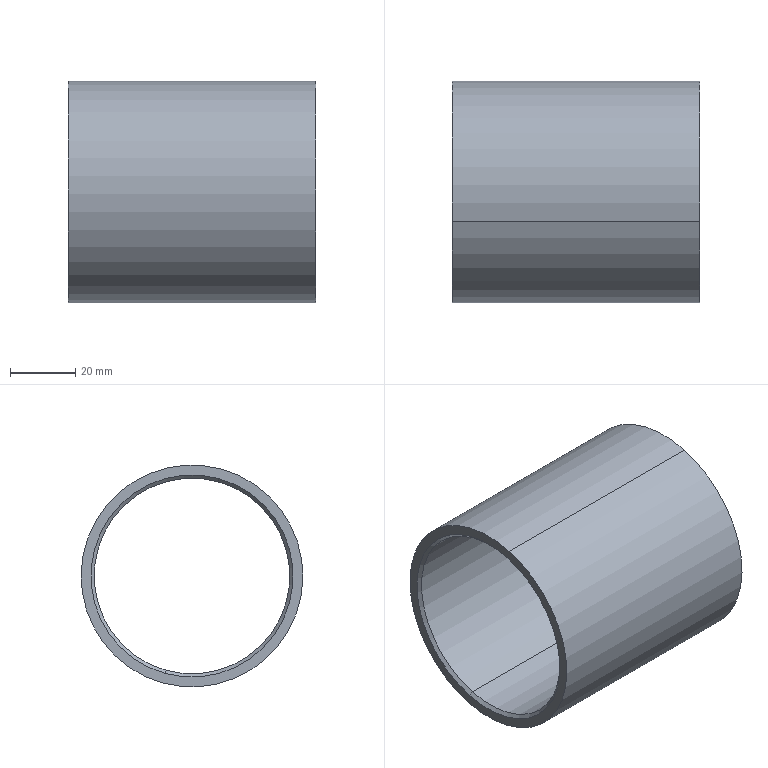Component | SolidWorks | SpindleSleeve3-1 | 1 solid | 10 faces | box 76 x 68 x 68 mm | volume 60932 mm3 | cone 4 | cylinder 4 | plane 2 | commonest cylinder face diameters 60 x2 68 x2
build123d program:
from build123d import *

# Parameters (mm, degrees)
SKETCH1_R           = 34
SKETCH1_R_2         = 30
BOSS_EXTRUDE1_DEPTH = 38
CHAMFER1_SIZE       = 1


with BuildPart() as part:
    # Sketch1 → Boss-Extrude1 (new, symmetric)
    with BuildSketch(Plane(origin=(0, 0, 0), x_dir=(1, 0, 0), z_dir=(0, 1, 0))):
        with Locations(Location((0, 0, 0), (0, 0, 270))):
            Circle(SKETCH1_R)
        with Locations(Location((0, 0, 0), (0, 0, 270))):
            Circle(SKETCH1_R_2, mode=Mode.SUBTRACT)
    extrude(amount=BOSS_EXTRUDE1_DEPTH, both=True)

    # Chamfer1
    chamfer1_edges = [part.edges().sort_by_distance(p)[0] for p in [
        (0, -38, -30),
        (0, 38, -30),
    ]]
    chamfer(chamfer1_edges, length=CHAMFER1_SIZE)


solid = part.part

# Placed as in the assembly
solid = solid.moved(Location((-713.197, 34.532, 0), (0, 0, 90)))
STEP:
#1=CARTESIAN_POINT('',(-26.622,1.671,-1.139));
#2=VERTEX_POINT('',#1);
#3=CARTESIAN_POINT('',(-26.622,1.048,1.139));
#4=VERTEX_POINT('',#3);
#5=CARTESIAN_POINT('',(-26.622,1.36,0.));
#6=DIRECTION('',(1.,0.,0.));
#7=DIRECTION('',(0.,0.2635,-0.9647));
#8=AXIS2_PLACEMENT_3D('',#5,#6,#7);
#9=CIRCLE('',#8,1.181);
#10=EDGE_CURVE('',#2,#4,#9,.T.);
#11=ORIENTED_EDGE('',*,*,#10,.F.);
#12=CARTESIAN_POINT('',(-26.583,1.681,-1.177));
#13=VERTEX_POINT('',#12);
#14=CARTESIAN_POINT('',(-26.583,1.681,-1.177));
#15=DIRECTION('',(0.7071,0.1863,-0.6821));
#16=VECTOR('',#15,39.37);
#17=LINE('',#14,#16);
#18=EDGE_CURVE('',#2,#13,#17,.T.);
#19=ORIENTED_EDGE('',*,*,#18,.T.);
#20=CARTESIAN_POINT('',(-26.583,1.038,1.177));
#21=VERTEX_POINT('',#20);
#22=CARTESIAN_POINT('',(-26.583,1.36,0.));
#23=DIRECTION('',(-1.,0.,0.));
#24=DIRECTION('',(0.,0.2635,-0.9647));
#25=AXIS2_PLACEMENT_3D('',#22,#23,#24);
#26=CIRCLE('',#25,1.22);
#27=EDGE_CURVE('',#21,#13,#26,.T.);
#28=ORIENTED_EDGE('',*,*,#27,.F.);
#29=CARTESIAN_POINT('',(-26.583,1.038,1.177));
#30=DIRECTION('',(0.7071,-0.1863,0.6821));
#31=VECTOR('',#30,39.37);
#32=LINE('',#29,#31);
#33=EDGE_CURVE('',#4,#21,#32,.T.);
#34=ORIENTED_EDGE('',*,*,#33,.F.);
#35=EDGE_LOOP('',(#11,#19,#28,#34));
#36=FACE_OUTER_BOUND('',#35,.T.);
#37=CARTESIAN_POINT('',(-26.583,1.36,0.));
#38=DIRECTION('',(1.,0.,0.));
#39=DIRECTION('',(0.,-0.2635,0.9647));
#40=AXIS2_PLACEMENT_3D('',#37,#38,#39);
#41=CONICAL_SURFACE('',#40,1.22,0.7854);
#42=ADVANCED_FACE('',(#36),#41,.F.);
#43=CARTESIAN_POINT('',(-29.535,1.048,1.139));
#44=VERTEX_POINT('',#43);
#45=CARTESIAN_POINT('',(-29.535,1.671,-1.139));
#46=VERTEX_POINT('',#45);
#47=CARTESIAN_POINT('',(-29.535,1.36,0.));
#48=DIRECTION('',(-1.,0.,0.));
#49=DIRECTION('',(0.,0.2635,-0.9647));
#50=AXIS2_PLACEMENT_3D('',#47,#48,#49);
#51=CIRCLE('',#50,1.181);
#52=EDGE_CURVE('',#44,#46,#51,.T.);
#53=ORIENTED_EDGE('',*,*,#52,.F.);
#54=CARTESIAN_POINT('',(-29.575,1.038,1.177));
#55=VERTEX_POINT('',#54);
#56=CARTESIAN_POINT('',(-29.535,1.048,1.139));
#57=DIRECTION('',(-0.7071,-0.1863,0.6821));
#58=VECTOR('',#57,39.37);
#59=LINE('',#56,#58);
#60=EDGE_CURVE('',#44,#55,#59,.T.);
#61=ORIENTED_EDGE('',*,*,#60,.T.);
#62=CARTESIAN_POINT('',(-29.575,1.681,-1.177));
#63=VERTEX_POINT('',#62);
#64=CARTESIAN_POINT('',(-29.575,1.36,0.));
#65=DIRECTION('',(1.,0.,0.));
#66=DIRECTION('',(0.,0.2635,-0.9647));
#67=AXIS2_PLACEMENT_3D('',#64,#65,#66);
#68=CIRCLE('',#67,1.22);
#69=EDGE_CURVE('',#63,#55,#68,.T.);
#70=ORIENTED_EDGE('',*,*,#69,.F.);
#71=CARTESIAN_POINT('',(-29.535,1.671,-1.139));
#72=DIRECTION('',(-0.7071,0.1863,-0.6821));
#73=VECTOR('',#72,39.37);
#74=LINE('',#71,#73);
#75=EDGE_CURVE('',#46,#63,#74,.T.);
#76=ORIENTED_EDGE('',*,*,#75,.F.);
#77=EDGE_LOOP('',(#53,#61,#70,#76));
#78=FACE_OUTER_BOUND('',#77,.T.);
#79=CARTESIAN_POINT('',(-29.535,1.36,0.));
#80=DIRECTION('',(-1.,0.,0.));
#81=DIRECTION('',(0.,0.2635,-0.9647));
#82=AXIS2_PLACEMENT_3D('',#79,#80,#81);
#83=CONICAL_SURFACE('',#82,1.181,0.7854);
#84=ADVANCED_FACE('',(#78),#83,.F.);
#85=ORIENTED_EDGE('',*,*,#52,.T.);
#86=CARTESIAN_POINT('',(-29.575,1.671,-1.139));
#87=DIRECTION('',(1.,0.,0.));
#88=VECTOR('',#87,39.37);
#89=LINE('',#86,#88);
#90=EDGE_CURVE('',#46,#2,#89,.T.);
#91=ORIENTED_EDGE('',*,*,#90,.T.);
#92=ORIENTED_EDGE('',*,*,#10,.T.);
#93=CARTESIAN_POINT('',(-29.575,1.048,1.139));
#94=DIRECTION('',(1.,0.,0.));
#95=VECTOR('',#94,39.37);
#96=LINE('',#93,#95);
#97=EDGE_CURVE('',#44,#4,#96,.T.);
#98=ORIENTED_EDGE('',*,*,#97,.F.);
#99=EDGE_LOOP('',(#85,#91,#92,#98));
#100=FACE_OUTER_BOUND('',#99,.T.);
#101=CARTESIAN_POINT('',(-29.575,1.36,0.));
#102=DIRECTION('',(1.,0.,0.));
#103=DIRECTION('',(0.,-0.2635,0.9647));
#104=AXIS2_PLACEMENT_3D('',#101,#102,#103);
#105=CYLINDRICAL_SURFACE('',#104,1.181);
#106=ADVANCED_FACE('',(#100),#105,.F.);
#107=CARTESIAN_POINT('',(-29.575,1.712,-1.291));
#108=VERTEX_POINT('',#107);
#109=CARTESIAN_POINT('',(-29.575,1.007,1.291));
#110=VERTEX_POINT('',#109);
#111=CARTESIAN_POINT('',(-29.575,1.36,0.));
#112=DIRECTION('',(-1.,0.,0.));
#113=DIRECTION('',(0.,0.2635,-0.9647));
#114=AXIS2_PLACEMENT_3D('',#111,#112,#113);
#115=CIRCLE('',#114,1.339);
#116=EDGE_CURVE('',#108,#110,#115,.T.);
#117=ORIENTED_EDGE('',*,*,#116,.F.);
#118=CARTESIAN_POINT('',(-26.583,1.712,-1.291));
#119=VERTEX_POINT('',#118);
#120=CARTESIAN_POINT('',(-29.575,1.712,-1.291));
#121=DIRECTION('',(1.,0.,0.));
#122=VECTOR('',#121,39.37);
#123=LINE('',#120,#122);
#124=EDGE_CURVE('',#108,#119,#123,.T.);
#125=ORIENTED_EDGE('',*,*,#124,.T.);
#126=CARTESIAN_POINT('',(-26.583,1.007,1.291));
#127=VERTEX_POINT('',#126);
#128=CARTESIAN_POINT('',(-26.583,1.36,0.));
#129=DIRECTION('',(-1.,0.,0.));
#130=DIRECTION('',(0.,0.2635,-0.9647));
#131=AXIS2_PLACEMENT_3D('',#128,#129,#130);
#132=CIRCLE('',#131,1.339);
#133=EDGE_CURVE('',#119,#127,#132,.T.);
#134=ORIENTED_EDGE('',*,*,#133,.T.);
#135=CARTESIAN_POINT('',(-29.575,1.007,1.291));
#136=DIRECTION('',(1.,0.,0.));
#137=VECTOR('',#136,39.37);
#138=LINE('',#135,#137);
#139=EDGE_CURVE('',#110,#127,#138,.T.);
#140=ORIENTED_EDGE('',*,*,#139,.F.);
#141=EDGE_LOOP('',(#117,#125,#134,#140));
#142=FACE_OUTER_BOUND('',#141,.T.);
#143=CARTESIAN_POINT('',(-29.575,1.36,0.));
#144=DIRECTION('',(1.,0.,0.));
#145=DIRECTION('',(0.,-0.2635,0.9647));
#146=AXIS2_PLACEMENT_3D('',#143,#144,#145);
#147=CYLINDRICAL_SURFACE('',#146,1.339);
#148=ADVANCED_FACE('',(#142),#147,.T.);
#149=ORIENTED_EDGE('',*,*,#69,.T.);
#150=CARTESIAN_POINT('',(-29.575,1.36,0.));
#151=DIRECTION('',(1.,0.,0.));
#152=DIRECTION('',(0.,0.2635,-0.9647));
#153=AXIS2_PLACEMENT_3D('',#150,#151,#152);
#154=CIRCLE('',#153,1.22);
#155=EDGE_CURVE('',#55,#63,#154,.T.);
#156=ORIENTED_EDGE('',*,*,#155,.T.);
#157=EDGE_LOOP('',(#149,#156));
#158=FACE_BOUND('',#157,.T.);
#159=CARTESIAN_POINT('',(-29.575,1.36,0.));
#160=DIRECTION('',(-1.,0.,0.));
#161=DIRECTION('',(0.,0.2635,-0.9647));
#162=AXIS2_PLACEMENT_3D('',#159,#160,#161);
#163=CIRCLE('',#162,1.339);
#164=EDGE_CURVE('',#110,#108,#163,.T.);
#165=ORIENTED_EDGE('',*,*,#164,.T.);
#166=ORIENTED_EDGE('',*,*,#116,.T.);
#167=EDGE_LOOP('',(#165,#166));
#168=FACE_OUTER_BOUND('',#167,.T.);
#169=CARTESIAN_POINT('',(-29.575,1.36,0.));
#170=DIRECTION('',(-1.,0.,0.));
#171=DIRECTION('',(0.,0.2635,-0.9647));
#172=AXIS2_PLACEMENT_3D('',#169,#170,#171);
#173=PLANE('',#172);
#174=ADVANCED_FACE('',(#158,#168),#173,.T.);
#175=ORIENTED_EDGE('',*,*,#27,.T.);
#176=CARTESIAN_POINT('',(-26.583,1.36,0.));
#177=DIRECTION('',(-1.,0.,0.));
#178=DIRECTION('',(0.,0.2635,-0.9647));
#179=AXIS2_PLACEMENT_3D('',#176,#177,#178);
#180=CIRCLE('',#179,1.22);
#181=EDGE_CURVE('',#13,#21,#180,.T.);
#182=ORIENTED_EDGE('',*,*,#181,.T.);
#183=EDGE_LOOP('',(#175,#182));
#184=FACE_BOUND('',#183,.T.);
#185=CARTESIAN_POINT('',(-26.583,1.36,0.));
#186=DIRECTION('',(-1.,0.,0.));
#187=DIRECTION('',(0.,0.2635,-0.9647));
#188=AXIS2_PLACEMENT_3D('',#185,#186,#187);
#189=CIRCLE('',#188,1.339);
#190=EDGE_CURVE('',#127,#119,#189,.T.);
#191=ORIENTED_EDGE('',*,*,#190,.F.);
#192=ORIENTED_EDGE('',*,*,#133,.F.);
#193=EDGE_LOOP('',(#191,#192));
#194=FACE_OUTER_BOUND('',#193,.T.);
#195=CARTESIAN_POINT('',(-26.583,1.36,0.));
#196=DIRECTION('',(-1.,0.,0.));
#197=DIRECTION('',(0.,0.2635,-0.9647));
#198=AXIS2_PLACEMENT_3D('',#195,#196,#197);
#199=PLANE('',#198);
#200=ADVANCED_FACE('',(#184,#194),#199,.F.);
#201=ORIENTED_EDGE('',*,*,#124,.F.);
#202=ORIENTED_EDGE('',*,*,#164,.F.);
#203=ORIENTED_EDGE('',*,*,#139,.T.);
#204=ORIENTED_EDGE('',*,*,#190,.T.);
#205=EDGE_LOOP('',(#201,#202,#203,#204));
#206=FACE_OUTER_BOUND('',#205,.T.);
#207=CARTESIAN_POINT('',(-29.575,1.36,0.));
#208=DIRECTION('',(1.,0.,0.));
#209=DIRECTION('',(0.,-0.2635,0.9647));
#210=AXIS2_PLACEMENT_3D('',#207,#208,#209);
#211=CYLINDRICAL_SURFACE('',#210,1.339);
#212=ADVANCED_FACE('',(#206),#211,.T.);
#213=ORIENTED_EDGE('',*,*,#90,.F.);
#214=CARTESIAN_POINT('',(-29.535,1.36,0.));
#215=DIRECTION('',(-1.,0.,0.));
#216=DIRECTION('',(0.,0.2635,-0.9647));
#217=AXIS2_PLACEMENT_3D('',#214,#215,#216);
#218=CIRCLE('',#217,1.181);
#219=EDGE_CURVE('',#46,#44,#218,.T.);
#220=ORIENTED_EDGE('',*,*,#219,.T.);
#221=ORIENTED_EDGE('',*,*,#97,.T.);
#222=CARTESIAN_POINT('',(-26.622,1.36,0.));
#223=DIRECTION('',(1.,0.,0.));
#224=DIRECTION('',(0.,0.2635,-0.9647));
#225=AXIS2_PLACEMENT_3D('',#222,#223,#224);
#226=CIRCLE('',#225,1.181);
#227=EDGE_CURVE('',#4,#2,#226,.T.);
#228=ORIENTED_EDGE('',*,*,#227,.T.);
#229=EDGE_LOOP('',(#213,#220,#221,#228));
#230=FACE_OUTER_BOUND('',#229,.T.);
#231=CARTESIAN_POINT('',(-29.575,1.36,0.));
#232=DIRECTION('',(1.,0.,0.));
#233=DIRECTION('',(0.,-0.2635,0.9647));
#234=AXIS2_PLACEMENT_3D('',#231,#232,#233);
#235=CYLINDRICAL_SURFACE('',#234,1.181);
#236=ADVANCED_FACE('',(#230),#235,.F.);
#237=ORIENTED_EDGE('',*,*,#60,.F.);
#238=ORIENTED_EDGE('',*,*,#219,.F.);
#239=ORIENTED_EDGE('',*,*,#75,.T.);
#240=ORIENTED_EDGE('',*,*,#155,.F.);
#241=EDGE_LOOP('',(#237,#238,#239,#240));
#242=FACE_OUTER_BOUND('',#241,.T.);
#243=CARTESIAN_POINT('',(-29.535,1.36,0.));
#244=DIRECTION('',(-1.,0.,0.));
#245=DIRECTION('',(0.,0.2635,-0.9647));
#246=AXIS2_PLACEMENT_3D('',#243,#244,#245);
#247=CONICAL_SURFACE('',#246,1.181,0.7854);
#248=ADVANCED_FACE('',(#242),#247,.F.);
#249=ORIENTED_EDGE('',*,*,#18,.F.);
#250=ORIENTED_EDGE('',*,*,#227,.F.);
#251=ORIENTED_EDGE('',*,*,#33,.T.);
#252=ORIENTED_EDGE('',*,*,#181,.F.);
#253=EDGE_LOOP('',(#249,#250,#251,#252));
#254=FACE_OUTER_BOUND('',#253,.T.);
#255=CARTESIAN_POINT('',(-26.583,1.36,0.));
#256=DIRECTION('',(1.,0.,0.));
#257=DIRECTION('',(0.,-0.2635,0.9647));
#258=AXIS2_PLACEMENT_3D('',#255,#256,#257);
#259=CONICAL_SURFACE('',#258,1.22,0.7854);
#260=ADVANCED_FACE('',(#254),#259,.F.);
#261=CLOSED_SHELL('',(#42,#84,#106,#148,#174,#200,#212,#236,#248,#260));
#262=MANIFOLD_SOLID_BREP('',#261);
#263=CARTESIAN_POINT('',(0.,0.,0.));
#264=DIRECTION('',(0.,0.,1.));
#265=DIRECTION('',(1.,0.,0.));
#266=AXIS2_PLACEMENT_3D('',#263,#264,#265);
#267=(LENGTH_UNIT()NAMED_UNIT(*)SI_UNIT($,.METRE.));
#268=LENGTH_MEASURE_WITH_UNIT(LENGTH_MEASURE(0.0254),#267);
#269=DIMENSIONAL_EXPONENTS(1.,0.,0.,0.,0.,0.,0.);
#270=(CONVERSION_BASED_UNIT('',#268)LENGTH_UNIT()NAMED_UNIT(#269));
#271=UNCERTAINTY_MEASURE_WITH_UNIT(LENGTH_MEASURE(0.00001),#270,'','');
#272=(NAMED_UNIT(*)PLANE_ANGLE_UNIT()SI_UNIT($,.RADIAN.));
#273=(NAMED_UNIT(*)SI_UNIT($,.STERADIAN.)SOLID_ANGLE_UNIT());
#274=(GEOMETRIC_REPRESENTATION_CONTEXT(3)GLOBAL_UNCERTAINTY_ASSIGNED_CONTEXT((#271))GLOBAL_UNIT_ASSIGNED_CONTEXT((#270,#272,#273))REPRESENTATION_CONTEXT('',''));
#275=ADVANCED_BREP_SHAPE_REPRESENTATION('',(#262,#266),#274);
#276=COLOUR_RGB('',0.7922,0.8196,0.9333);
#277=FILL_AREA_STYLE_COLOUR('',#276);
#278=FILL_AREA_STYLE('',(#277));
#279=SURFACE_STYLE_FILL_AREA(#278);
#280=SURFACE_SIDE_STYLE('',(#279));
#281=SURFACE_STYLE_USAGE(.BOTH.,#280);
#282=PRESENTATION_STYLE_ASSIGNMENT((#281));
#283=STYLED_ITEM('',(#282),#262);
#284=PRESENTATION_LAYER_ASSIGNMENT('','',(#283));
#285=(LENGTH_UNIT()NAMED_UNIT(*)SI_UNIT($,.METRE.));
#286=LENGTH_MEASURE_WITH_UNIT(LENGTH_MEASURE(0.0254),#285);
#287=DIMENSIONAL_EXPONENTS(1.,0.,0.,0.,0.,0.,0.);
#288=(CONVERSION_BASED_UNIT('',#286)LENGTH_UNIT()NAMED_UNIT(#287));
#289=UNCERTAINTY_MEASURE_WITH_UNIT(LENGTH_MEASURE(0.00001),#288,'','');
#290=(NAMED_UNIT(*)PLANE_ANGLE_UNIT()SI_UNIT($,.RADIAN.));
#291=(NAMED_UNIT(*)SI_UNIT($,.STERADIAN.)SOLID_ANGLE_UNIT());
#292=(GEOMETRIC_REPRESENTATION_CONTEXT(3)GLOBAL_UNCERTAINTY_ASSIGNED_CONTEXT((#289))GLOBAL_UNIT_ASSIGNED_CONTEXT((#288,#290,#291))REPRESENTATION_CONTEXT('',''));
#293=MECHANICAL_DESIGN_GEOMETRIC_PRESENTATION_REPRESENTATION('',(#283),#292);